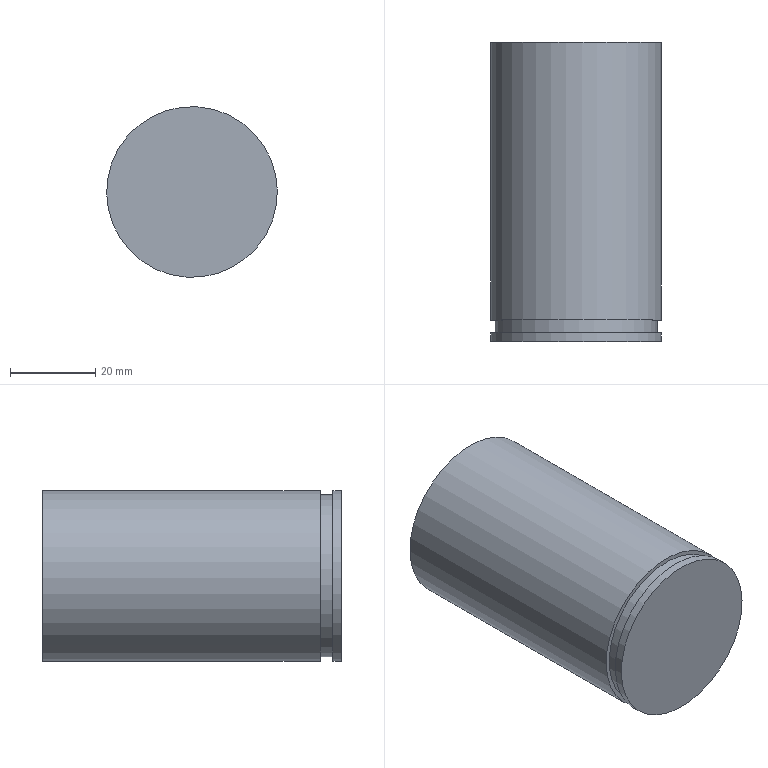Component | NX | MODEL5 | 1 solid | 10 faces | box 40 x 70 x 40 mm | volume 59821 mm3 | cylinder 4 | plane 4 | cone 2 | commonest cylinder face diameters 40 x2 25 x1 38 x1
STEP:
#1=CARTESIAN_POINT('',(0.,0.,0.));
#2=DIRECTION('',(0.,0.,1.));
#3=DIRECTION('',(1.,0.,0.));
#4=AXIS2_PLACEMENT_3D('',#1,#2,#3);
#5=CARTESIAN_POINT('',(18.481,-498.,7.646));
#6=VERTEX_POINT('',#5);
#7=CARTESIAN_POINT('',(-18.481,-498.,-7.646));
#8=VERTEX_POINT('',#7);
#9=CARTESIAN_POINT('',(0.,-498.,0.));
#10=DIRECTION('',(0.,1.,0.));
#11=DIRECTION('',(-0.924,0.,-0.3823));
#12=AXIS2_PLACEMENT_3D('',#9,#10,#11);
#13=CIRCLE('',#12,20.);
#14=CARTESIAN_POINT('',(0.,-568.,0.));
#15=DIRECTION('',(0.,1.,0.));
#16=DIRECTION('',(0.924,0.,0.3823));
#17=AXIS2_PLACEMENT_3D('',#14,#15,#16);
#18=CYLINDRICAL_SURFACE('',#17,20.);
#19=CARTESIAN_POINT('',(-3.142,70.));
#20=DIRECTION('',(1.,0.));
#21=VECTOR('',#20,1.);
#22=LINE('',#19,#21);
#23=(GEOMETRIC_REPRESENTATION_CONTEXT(2)PARAMETRIC_REPRESENTATION_CONTEXT()REPRESENTATION_CONTEXT('',''));
#24=DEFINITIONAL_REPRESENTATION('',(#22),#23);
#25=PCURVE('',#18,#24);
#26=CARTESIAN_POINT('',(0.,-498.,0.));
#27=DIRECTION('',(0.,1.,0.));
#28=DIRECTION('',(0.924,0.,0.3823));
#29=AXIS2_PLACEMENT_3D('',#26,#27,#28);
#30=PLANE('',#29);
#31=CARTESIAN_POINT('',(0.,0.));
#32=DIRECTION('',(-1.,0.));
#33=AXIS2_PLACEMENT_2D('',#31,#32);
#34=CIRCLE('',#33,20.);
#35=(GEOMETRIC_REPRESENTATION_CONTEXT(2)PARAMETRIC_REPRESENTATION_CONTEXT()REPRESENTATION_CONTEXT('',''));
#36=DEFINITIONAL_REPRESENTATION('',(#34),#35);
#37=PCURVE('',#30,#36);
#38=SURFACE_CURVE('',#13,(#25,#37),.PCURVE_S1.);
#39=EDGE_CURVE('',#6,#8,#38,.T.);
#40=ORIENTED_EDGE('',*,*,#39,.F.);
#41=CARTESIAN_POINT('',(18.481,-563.,7.646));
#42=VERTEX_POINT('',#41);
#43=CARTESIAN_POINT('',(18.481,-563.,7.646));
#44=CARTESIAN_POINT('',(18.481,-498.,7.646));
#45=B_SPLINE_CURVE_WITH_KNOTS('',1,(#43,#44),.UNSPECIFIED.,.F.,.F.,(2,2),(5.,70.),.PIECEWISE_BEZIER_KNOTS.);
#46=CARTESIAN_POINT('',(0.,0.));
#47=DIRECTION('',(0.,1.));
#48=VECTOR('',#47,1.);
#49=LINE('',#46,#48);
#50=(GEOMETRIC_REPRESENTATION_CONTEXT(2)PARAMETRIC_REPRESENTATION_CONTEXT()REPRESENTATION_CONTEXT('',''));
#51=DEFINITIONAL_REPRESENTATION('',(#49),#50);
#52=PCURVE('',#18,#51);
#53=CARTESIAN_POINT('',(6.283,0.));
#54=DIRECTION('',(0.,1.));
#55=VECTOR('',#54,1.);
#56=LINE('',#53,#55);
#57=(GEOMETRIC_REPRESENTATION_CONTEXT(2)PARAMETRIC_REPRESENTATION_CONTEXT()REPRESENTATION_CONTEXT('',''));
#58=DEFINITIONAL_REPRESENTATION('',(#56),#57);
#59=PCURVE('',#18,#58);
#60=SEAM_CURVE('',#45,(#52,#59),.PCURVE_S1.);
#61=EDGE_CURVE('',#42,#6,#60,.T.);
#62=ORIENTED_EDGE('',*,*,#61,.F.);
#63=CARTESIAN_POINT('',(0.,-563.,0.));
#64=DIRECTION('',(0.,1.,0.));
#65=DIRECTION('',(0.924,0.,0.3823));
#66=AXIS2_PLACEMENT_3D('',#63,#64,#65);
#67=CIRCLE('',#66,20.);
#68=CARTESIAN_POINT('',(0.,5.));
#69=DIRECTION('',(1.,0.));
#70=VECTOR('',#69,1.);
#71=LINE('',#68,#70);
#72=(GEOMETRIC_REPRESENTATION_CONTEXT(2)PARAMETRIC_REPRESENTATION_CONTEXT()REPRESENTATION_CONTEXT('',''));
#73=DEFINITIONAL_REPRESENTATION('',(#71),#72);
#74=PCURVE('',#18,#73);
#75=CARTESIAN_POINT('',(-18.481,-563.,-7.646));
#76=DIRECTION('',(0.,-1.,0.));
#77=DIRECTION('',(-0.924,0.,-0.3823));
#78=AXIS2_PLACEMENT_3D('',#75,#76,#77);
#79=PLANE('',#78);
#80=CARTESIAN_POINT('',(-40.,-0.));
#81=CARTESIAN_POINT('',(-40.,34.641));
#82=CARTESIAN_POINT('',(-10.,17.321));
#83=CARTESIAN_POINT('',(20.,-0.));
#84=CARTESIAN_POINT('',(-10.,-17.321));
#85=CARTESIAN_POINT('',(-40.,-34.641));
#86=CARTESIAN_POINT('',(-40.,-0.));
#87=(BOUNDED_CURVE()B_SPLINE_CURVE(2,(#80,#81,#82,#83,#84,#85,#86),.UNSPECIFIED.,.T.,.F.)B_SPLINE_CURVE_WITH_KNOTS((1,2,2,2,2,1),(-2.094,0.,2.094,4.189,6.283,8.378),.UNSPECIFIED.)CURVE()GEOMETRIC_REPRESENTATION_ITEM()RATIONAL_B_SPLINE_CURVE((1.,0.5,1.,0.5,1.,0.5,1.))REPRESENTATION_ITEM(''));
#88=(GEOMETRIC_REPRESENTATION_CONTEXT(2)PARAMETRIC_REPRESENTATION_CONTEXT()REPRESENTATION_CONTEXT('',''));
#89=DEFINITIONAL_REPRESENTATION('',(#87),#88);
#90=PCURVE('',#79,#89);
#91=SURFACE_CURVE('',#67,(#74,#90),.PCURVE_S1.);
#92=EDGE_CURVE('',#42,#42,#91,.T.);
#93=ORIENTED_EDGE('',*,*,#92,.T.);
#94=ORIENTED_EDGE('',*,*,#61,.T.);
#95=CARTESIAN_POINT('',(0.,-498.,0.));
#96=DIRECTION('',(0.,1.,0.));
#97=DIRECTION('',(-0.924,0.,-0.3823));
#98=AXIS2_PLACEMENT_3D('',#95,#96,#97);
#99=CIRCLE('',#98,20.);
#100=CARTESIAN_POINT('',(3.142,70.));
#101=DIRECTION('',(1.,0.));
#102=VECTOR('',#101,1.);
#103=LINE('',#100,#102);
#104=(GEOMETRIC_REPRESENTATION_CONTEXT(2)PARAMETRIC_REPRESENTATION_CONTEXT()REPRESENTATION_CONTEXT('',''));
#105=DEFINITIONAL_REPRESENTATION('',(#103),#104);
#106=PCURVE('',#18,#105);
#107=CARTESIAN_POINT('',(0.,0.));
#108=DIRECTION('',(-1.,0.));
#109=AXIS2_PLACEMENT_2D('',#107,#108);
#110=CIRCLE('',#109,20.);
#111=(GEOMETRIC_REPRESENTATION_CONTEXT(2)PARAMETRIC_REPRESENTATION_CONTEXT()REPRESENTATION_CONTEXT('',''));
#112=DEFINITIONAL_REPRESENTATION('',(#110),#111);
#113=PCURVE('',#30,#112);
#114=SURFACE_CURVE('',#99,(#106,#113),.PCURVE_S1.);
#115=EDGE_CURVE('',#8,#6,#114,.T.);
#116=ORIENTED_EDGE('',*,*,#115,.F.);
#117=EDGE_LOOP('',(#40,#62,#93,#94,#116));
#118=FACE_BOUND('',#117,.T.);
#119=ADVANCED_FACE('',(#118),#18,.T.);
#120=CARTESIAN_POINT('',(12.474,-498.,5.161));
#121=VERTEX_POINT('',#120);
#122=CARTESIAN_POINT('',(0.,-498.,0.));
#123=DIRECTION('',(0.,-1.,0.));
#124=DIRECTION('',(0.924,0.,0.3823));
#125=AXIS2_PLACEMENT_3D('',#122,#123,#124);
#126=CIRCLE('',#125,13.5);
#127=CARTESIAN_POINT('',(13.5,0.));
#128=CARTESIAN_POINT('',(13.5,-23.383));
#129=CARTESIAN_POINT('',(-6.75,-11.691));
#130=CARTESIAN_POINT('',(-27.,-0.));
#131=CARTESIAN_POINT('',(-6.75,11.691));
#132=CARTESIAN_POINT('',(13.5,23.383));
#133=CARTESIAN_POINT('',(13.5,0.));
#134=(BOUNDED_CURVE()B_SPLINE_CURVE(2,(#127,#128,#129,#130,#131,#132,#133),.UNSPECIFIED.,.T.,.F.)B_SPLINE_CURVE_WITH_KNOTS((1,2,2,2,2,1),(-2.094,0.,2.094,4.189,6.283,8.378),.UNSPECIFIED.)CURVE()GEOMETRIC_REPRESENTATION_ITEM()RATIONAL_B_SPLINE_CURVE((1.,0.5,1.,0.5,1.,0.5,1.))REPRESENTATION_ITEM(''));
#135=(GEOMETRIC_REPRESENTATION_CONTEXT(2)PARAMETRIC_REPRESENTATION_CONTEXT()REPRESENTATION_CONTEXT('',''));
#136=DEFINITIONAL_REPRESENTATION('',(#134),#135);
#137=PCURVE('',#30,#136);
#138=CARTESIAN_POINT('',(0.,-498.,0.));
#139=DIRECTION('',(0.,1.,0.));
#140=DIRECTION('',(0.924,0.,0.3823));
#141=AXIS2_PLACEMENT_3D('',#138,#139,#140);
#142=CONICAL_SURFACE('',#141,13.5,0.7854);
#143=CARTESIAN_POINT('',(6.283,0.));
#144=DIRECTION('',(-1.,0.));
#145=VECTOR('',#144,1.);
#146=LINE('',#143,#145);
#147=(GEOMETRIC_REPRESENTATION_CONTEXT(2)PARAMETRIC_REPRESENTATION_CONTEXT()REPRESENTATION_CONTEXT('',''));
#148=DEFINITIONAL_REPRESENTATION('',(#146),#147);
#149=PCURVE('',#142,#148);
#150=SURFACE_CURVE('',#126,(#137,#149),.PCURVE_S1.);
#151=EDGE_CURVE('',#121,#121,#150,.T.);
#152=ORIENTED_EDGE('',*,*,#151,.T.);
#153=EDGE_LOOP('',(#152));
#154=FACE_BOUND('',#153,.T.);
#155=ORIENTED_EDGE('',*,*,#115,.T.);
#156=ORIENTED_EDGE('',*,*,#39,.T.);
#157=EDGE_LOOP('',(#155,#156));
#158=FACE_BOUND('',#157,.T.);
#159=ADVANCED_FACE('',(#154,#158),#30,.T.);
#160=CARTESIAN_POINT('',(-11.55,-552.,-4.779));
#161=VERTEX_POINT('',#160);
#162=CARTESIAN_POINT('',(11.55,-552.,4.779));
#163=VERTEX_POINT('',#162);
#164=CARTESIAN_POINT('',(0.,-552.,0.));
#165=DIRECTION('',(0.,-1.,0.));
#166=DIRECTION('',(-0.924,0.,-0.3823));
#167=AXIS2_PLACEMENT_3D('',#164,#165,#166);
#168=CIRCLE('',#167,12.5);
#169=CARTESIAN_POINT('',(0.,-552.,0.));
#170=DIRECTION('',(0.,1.,0.));
#171=DIRECTION('',(0.924,0.,0.3823));
#172=AXIS2_PLACEMENT_3D('',#169,#170,#171);
#173=CONICAL_SURFACE('',#172,12.5,1.03);
#174=CARTESIAN_POINT('',(3.142,0.));
#175=DIRECTION('',(-1.,0.));
#176=VECTOR('',#175,1.);
#177=LINE('',#174,#176);
#178=(GEOMETRIC_REPRESENTATION_CONTEXT(2)PARAMETRIC_REPRESENTATION_CONTEXT()REPRESENTATION_CONTEXT('',''));
#179=DEFINITIONAL_REPRESENTATION('',(#177),#178);
#180=PCURVE('',#173,#179);
#181=CARTESIAN_POINT('',(0.,-498.,0.));
#182=DIRECTION('',(0.,-1.,0.));
#183=DIRECTION('',(-0.924,0.,-0.3823));
#184=AXIS2_PLACEMENT_3D('',#181,#182,#183);
#185=CYLINDRICAL_SURFACE('',#184,12.5);
#186=CARTESIAN_POINT('',(6.283,54.));
#187=DIRECTION('',(1.,0.));
#188=VECTOR('',#187,1.);
#189=LINE('',#186,#188);
#190=(GEOMETRIC_REPRESENTATION_CONTEXT(2)PARAMETRIC_REPRESENTATION_CONTEXT()REPRESENTATION_CONTEXT('',''));
#191=DEFINITIONAL_REPRESENTATION('',(#189),#190);
#192=PCURVE('',#185,#191);
#193=SURFACE_CURVE('',#168,(#180,#192),.PCURVE_S1.);
#194=EDGE_CURVE('',#161,#163,#193,.T.);
#195=ORIENTED_EDGE('',*,*,#194,.T.);
#196=CARTESIAN_POINT('',(0.,-559.511,0.));
#197=VERTEX_POINT('',#196);
#198=CARTESIAN_POINT('',(0.,-559.511,0.));
#199=CARTESIAN_POINT('',(11.55,-552.,4.779));
#200=B_SPLINE_CURVE_WITH_KNOTS('',1,(#198,#199),.UNSPECIFIED.,.F.,.F.,(2,2),(-14.583,0.),.PIECEWISE_BEZIER_KNOTS.);
#201=CARTESIAN_POINT('',(0.,0.));
#202=DIRECTION('',(0.,1.));
#203=VECTOR('',#202,1.);
#204=LINE('',#201,#203);
#205=(GEOMETRIC_REPRESENTATION_CONTEXT(2)PARAMETRIC_REPRESENTATION_CONTEXT()REPRESENTATION_CONTEXT('',''));
#206=DEFINITIONAL_REPRESENTATION('',(#204),#205);
#207=PCURVE('',#173,#206);
#208=CARTESIAN_POINT('',(6.283,0.));
#209=DIRECTION('',(0.,1.));
#210=VECTOR('',#209,1.);
#211=LINE('',#208,#210);
#212=(GEOMETRIC_REPRESENTATION_CONTEXT(2)PARAMETRIC_REPRESENTATION_CONTEXT()REPRESENTATION_CONTEXT('',''));
#213=DEFINITIONAL_REPRESENTATION('',(#211),#212);
#214=PCURVE('',#173,#213);
#215=SEAM_CURVE('',#200,(#207,#214),.PCURVE_S1.);
#216=EDGE_CURVE('',#197,#163,#215,.T.);
#217=ORIENTED_EDGE('',*,*,#216,.F.);
#218=ORIENTED_EDGE('',*,*,#216,.T.);
#219=CARTESIAN_POINT('',(0.,-552.,0.));
#220=DIRECTION('',(0.,-1.,0.));
#221=DIRECTION('',(-0.924,0.,-0.3823));
#222=AXIS2_PLACEMENT_3D('',#219,#220,#221);
#223=CIRCLE('',#222,12.5);
#224=CARTESIAN_POINT('',(9.425,0.));
#225=DIRECTION('',(-1.,0.));
#226=VECTOR('',#225,1.);
#227=LINE('',#224,#226);
#228=(GEOMETRIC_REPRESENTATION_CONTEXT(2)PARAMETRIC_REPRESENTATION_CONTEXT()REPRESENTATION_CONTEXT('',''));
#229=DEFINITIONAL_REPRESENTATION('',(#227),#228);
#230=PCURVE('',#173,#229);
#231=CARTESIAN_POINT('',(0.,54.));
#232=DIRECTION('',(1.,0.));
#233=VECTOR('',#232,1.);
#234=LINE('',#231,#233);
#235=(GEOMETRIC_REPRESENTATION_CONTEXT(2)PARAMETRIC_REPRESENTATION_CONTEXT()REPRESENTATION_CONTEXT('',''));
#236=DEFINITIONAL_REPRESENTATION('',(#234),#235);
#237=PCURVE('',#185,#236);
#238=SURFACE_CURVE('',#223,(#230,#237),.PCURVE_S1.);
#239=EDGE_CURVE('',#163,#161,#238,.T.);
#240=ORIENTED_EDGE('',*,*,#239,.T.);
#241=EDGE_LOOP('',(#195,#217,#218,#240));
#242=FACE_BOUND('',#241,.F.);
#243=ADVANCED_FACE('',(#242),#173,.F.);
#244=CARTESIAN_POINT('',(11.55,-499.,4.779));
#245=VERTEX_POINT('',#244);
#246=CARTESIAN_POINT('',(0.,-499.,0.));
#247=DIRECTION('',(0.,1.,0.));
#248=DIRECTION('',(0.924,0.,0.3823));
#249=AXIS2_PLACEMENT_3D('',#246,#247,#248);
#250=CIRCLE('',#249,12.5);
#251=CARTESIAN_POINT('',(9.425,1.));
#252=DIRECTION('',(-1.,0.));
#253=VECTOR('',#252,1.);
#254=LINE('',#251,#253);
#255=(GEOMETRIC_REPRESENTATION_CONTEXT(2)PARAMETRIC_REPRESENTATION_CONTEXT()REPRESENTATION_CONTEXT('',''));
#256=DEFINITIONAL_REPRESENTATION('',(#254),#255);
#257=PCURVE('',#185,#256);
#258=CARTESIAN_POINT('',(0.,-1.));
#259=DIRECTION('',(1.,-0.));
#260=VECTOR('',#259,1.);
#261=LINE('',#258,#260);
#262=(GEOMETRIC_REPRESENTATION_CONTEXT(2)PARAMETRIC_REPRESENTATION_CONTEXT()REPRESENTATION_CONTEXT('',''));
#263=DEFINITIONAL_REPRESENTATION('',(#261),#262);
#264=PCURVE('',#142,#263);
#265=SURFACE_CURVE('',#250,(#257,#264),.PCURVE_S1.);
#266=EDGE_CURVE('',#245,#245,#265,.T.);
#267=ORIENTED_EDGE('',*,*,#266,.F.);
#268=CARTESIAN_POINT('',(11.55,-499.,4.779));
#269=CARTESIAN_POINT('',(11.55,-552.,4.779));
#270=B_SPLINE_CURVE_WITH_KNOTS('',1,(#268,#269),.UNSPECIFIED.,.F.,.F.,(2,2),(1.,54.),.PIECEWISE_BEZIER_KNOTS.);
#271=CARTESIAN_POINT('',(9.425,0.));
#272=DIRECTION('',(0.,1.));
#273=VECTOR('',#272,1.);
#274=LINE('',#271,#273);
#275=(GEOMETRIC_REPRESENTATION_CONTEXT(2)PARAMETRIC_REPRESENTATION_CONTEXT()REPRESENTATION_CONTEXT('',''));
#276=DEFINITIONAL_REPRESENTATION('',(#274),#275);
#277=PCURVE('',#185,#276);
#278=CARTESIAN_POINT('',(3.142,0.));
#279=DIRECTION('',(0.,1.));
#280=VECTOR('',#279,1.);
#281=LINE('',#278,#280);
#282=(GEOMETRIC_REPRESENTATION_CONTEXT(2)PARAMETRIC_REPRESENTATION_CONTEXT()REPRESENTATION_CONTEXT('',''));
#283=DEFINITIONAL_REPRESENTATION('',(#281),#282);
#284=PCURVE('',#185,#283);
#285=SEAM_CURVE('',#270,(#277,#284),.PCURVE_S1.);
#286=EDGE_CURVE('',#245,#163,#285,.T.);
#287=ORIENTED_EDGE('',*,*,#286,.T.);
#288=ORIENTED_EDGE('',*,*,#194,.F.);
#289=ORIENTED_EDGE('',*,*,#239,.F.);
#290=ORIENTED_EDGE('',*,*,#286,.F.);
#291=EDGE_LOOP('',(#267,#287,#288,#289,#290));
#292=FACE_BOUND('',#291,.F.);
#293=ADVANCED_FACE('',(#292),#185,.F.);
#294=ORIENTED_EDGE('',*,*,#266,.T.);
#295=CARTESIAN_POINT('',(11.55,-499.,4.779));
#296=CARTESIAN_POINT('',(12.474,-498.,5.161));
#297=B_SPLINE_CURVE_WITH_KNOTS('',1,(#295,#296),.UNSPECIFIED.,.F.,.F.,(2,2),(-1.414,0.),.PIECEWISE_BEZIER_KNOTS.);
#298=CARTESIAN_POINT('',(6.283,0.));
#299=DIRECTION('',(0.,1.));
#300=VECTOR('',#299,1.);
#301=LINE('',#298,#300);
#302=(GEOMETRIC_REPRESENTATION_CONTEXT(2)PARAMETRIC_REPRESENTATION_CONTEXT()REPRESENTATION_CONTEXT('',''));
#303=DEFINITIONAL_REPRESENTATION('',(#301),#302);
#304=PCURVE('',#142,#303);
#305=CARTESIAN_POINT('',(0.,0.));
#306=DIRECTION('',(0.,1.));
#307=VECTOR('',#306,1.);
#308=LINE('',#305,#307);
#309=(GEOMETRIC_REPRESENTATION_CONTEXT(2)PARAMETRIC_REPRESENTATION_CONTEXT()REPRESENTATION_CONTEXT('',''));
#310=DEFINITIONAL_REPRESENTATION('',(#308),#309);
#311=PCURVE('',#142,#310);
#312=SEAM_CURVE('',#297,(#304,#311),.PCURVE_S1.);
#313=EDGE_CURVE('',#245,#121,#312,.T.);
#314=ORIENTED_EDGE('',*,*,#313,.T.);
#315=ORIENTED_EDGE('',*,*,#151,.T.);
#316=ORIENTED_EDGE('',*,*,#313,.F.);
#317=EDGE_LOOP('',(#294,#314,#315,#316));
#318=FACE_BOUND('',#317,.F.);
#319=ADVANCED_FACE('',(#318),#142,.F.);
#320=CARTESIAN_POINT('',(17.557,-563.,7.264));
#321=VERTEX_POINT('',#320);
#322=CARTESIAN_POINT('',(0.,-563.,0.));
#323=DIRECTION('',(0.,1.,0.));
#324=DIRECTION('',(0.924,0.,0.3823));
#325=AXIS2_PLACEMENT_3D('',#322,#323,#324);
#326=CIRCLE('',#325,19.);
#327=CARTESIAN_POINT('',(-39.,-0.));
#328=CARTESIAN_POINT('',(-39.,32.909));
#329=CARTESIAN_POINT('',(-10.5,16.454));
#330=CARTESIAN_POINT('',(18.,-0.));
#331=CARTESIAN_POINT('',(-10.5,-16.454));
#332=CARTESIAN_POINT('',(-39.,-32.909));
#333=CARTESIAN_POINT('',(-39.,-0.));
#334=(BOUNDED_CURVE()B_SPLINE_CURVE(2,(#327,#328,#329,#330,#331,#332,#333),.UNSPECIFIED.,.T.,.F.)B_SPLINE_CURVE_WITH_KNOTS((1,2,2,2,2,1),(-2.094,0.,2.094,4.189,6.283,8.378),.UNSPECIFIED.)CURVE()GEOMETRIC_REPRESENTATION_ITEM()RATIONAL_B_SPLINE_CURVE((1.,0.5,1.,0.5,1.,0.5,1.))REPRESENTATION_ITEM(''));
#335=(GEOMETRIC_REPRESENTATION_CONTEXT(2)PARAMETRIC_REPRESENTATION_CONTEXT()REPRESENTATION_CONTEXT('',''));
#336=DEFINITIONAL_REPRESENTATION('',(#334),#335);
#337=PCURVE('',#79,#336);
#338=CARTESIAN_POINT('',(0.,-498.,0.));
#339=DIRECTION('',(0.,1.,0.));
#340=DIRECTION('',(0.924,0.,0.3823));
#341=AXIS2_PLACEMENT_3D('',#338,#339,#340);
#342=CYLINDRICAL_SURFACE('',#341,19.);
#343=CARTESIAN_POINT('',(0.,-65.));
#344=DIRECTION('',(1.,0.));
#345=VECTOR('',#344,1.);
#346=LINE('',#343,#345);
#347=(GEOMETRIC_REPRESENTATION_CONTEXT(2)PARAMETRIC_REPRESENTATION_CONTEXT()REPRESENTATION_CONTEXT('',''));
#348=DEFINITIONAL_REPRESENTATION('',(#346),#347);
#349=PCURVE('',#342,#348);
#350=SURFACE_CURVE('',#326,(#337,#349),.PCURVE_S1.);
#351=EDGE_CURVE('',#321,#321,#350,.T.);
#352=ORIENTED_EDGE('',*,*,#351,.T.);
#353=EDGE_LOOP('',(#352));
#354=FACE_BOUND('',#353,.T.);
#355=ORIENTED_EDGE('',*,*,#92,.F.);
#356=EDGE_LOOP('',(#355));
#357=FACE_BOUND('',#356,.T.);
#358=ADVANCED_FACE('',(#354,#357),#79,.T.);
#359=CARTESIAN_POINT('',(17.557,-566.,7.264));
#360=VERTEX_POINT('',#359);
#361=CARTESIAN_POINT('',(0.,-566.,0.));
#362=DIRECTION('',(0.,1.,0.));
#363=DIRECTION('',(0.924,0.,0.3823));
#364=AXIS2_PLACEMENT_3D('',#361,#362,#363);
#365=CIRCLE('',#364,19.);
#366=CARTESIAN_POINT('',(0.,-68.));
#367=DIRECTION('',(1.,0.));
#368=VECTOR('',#367,1.);
#369=LINE('',#366,#368);
#370=(GEOMETRIC_REPRESENTATION_CONTEXT(2)PARAMETRIC_REPRESENTATION_CONTEXT()REPRESENTATION_CONTEXT('',''));
#371=DEFINITIONAL_REPRESENTATION('',(#369),#370);
#372=PCURVE('',#342,#371);
#373=CARTESIAN_POINT('',(-17.557,-566.,-7.264));
#374=DIRECTION('',(0.,1.,0.));
#375=DIRECTION('',(0.924,0.,0.3823));
#376=AXIS2_PLACEMENT_3D('',#373,#374,#375);
#377=PLANE('',#376);
#378=CARTESIAN_POINT('',(19.,0.));
#379=DIRECTION('',(1.,0.));
#380=AXIS2_PLACEMENT_2D('',#378,#379);
#381=CIRCLE('',#380,19.);
#382=(GEOMETRIC_REPRESENTATION_CONTEXT(2)PARAMETRIC_REPRESENTATION_CONTEXT()REPRESENTATION_CONTEXT('',''));
#383=DEFINITIONAL_REPRESENTATION('',(#381),#382);
#384=PCURVE('',#377,#383);
#385=SURFACE_CURVE('',#365,(#372,#384),.PCURVE_S1.);
#386=EDGE_CURVE('',#360,#360,#385,.T.);
#387=ORIENTED_EDGE('',*,*,#386,.T.);
#388=CARTESIAN_POINT('',(17.557,-566.,7.264));
#389=CARTESIAN_POINT('',(17.557,-563.,7.264));
#390=B_SPLINE_CURVE_WITH_KNOTS('',1,(#388,#389),.UNSPECIFIED.,.F.,.F.,(2,2),(-68.,-65.),.PIECEWISE_BEZIER_KNOTS.);
#391=CARTESIAN_POINT('',(6.283,0.));
#392=DIRECTION('',(0.,1.));
#393=VECTOR('',#392,1.);
#394=LINE('',#391,#393);
#395=(GEOMETRIC_REPRESENTATION_CONTEXT(2)PARAMETRIC_REPRESENTATION_CONTEXT()REPRESENTATION_CONTEXT('',''));
#396=DEFINITIONAL_REPRESENTATION('',(#394),#395);
#397=PCURVE('',#342,#396);
#398=CARTESIAN_POINT('',(0.,0.));
#399=DIRECTION('',(0.,1.));
#400=VECTOR('',#399,1.);
#401=LINE('',#398,#400);
#402=(GEOMETRIC_REPRESENTATION_CONTEXT(2)PARAMETRIC_REPRESENTATION_CONTEXT()REPRESENTATION_CONTEXT('',''));
#403=DEFINITIONAL_REPRESENTATION('',(#401),#402);
#404=PCURVE('',#342,#403);
#405=SEAM_CURVE('',#390,(#397,#404),.PCURVE_S1.);
#406=EDGE_CURVE('',#360,#321,#405,.T.);
#407=ORIENTED_EDGE('',*,*,#406,.T.);
#408=ORIENTED_EDGE('',*,*,#351,.F.);
#409=ORIENTED_EDGE('',*,*,#406,.F.);
#410=EDGE_LOOP('',(#387,#407,#408,#409));
#411=FACE_BOUND('',#410,.T.);
#412=ADVANCED_FACE('',(#411),#342,.T.);
#413=CARTESIAN_POINT('',(18.481,-566.,7.646));
#414=VERTEX_POINT('',#413);
#415=CARTESIAN_POINT('',(0.,-566.,0.));
#416=DIRECTION('',(0.,1.,0.));
#417=DIRECTION('',(0.924,0.,0.3823));
#418=AXIS2_PLACEMENT_3D('',#415,#416,#417);
#419=CIRCLE('',#418,20.);
#420=CARTESIAN_POINT('',(19.,0.));
#421=DIRECTION('',(1.,0.));
#422=AXIS2_PLACEMENT_2D('',#420,#421);
#423=CIRCLE('',#422,20.);
#424=(GEOMETRIC_REPRESENTATION_CONTEXT(2)PARAMETRIC_REPRESENTATION_CONTEXT()REPRESENTATION_CONTEXT('',''));
#425=DEFINITIONAL_REPRESENTATION('',(#423),#424);
#426=PCURVE('',#377,#425);
#427=CARTESIAN_POINT('',(0.,-568.,0.));
#428=DIRECTION('',(0.,1.,0.));
#429=DIRECTION('',(0.924,0.,0.3823));
#430=AXIS2_PLACEMENT_3D('',#427,#428,#429);
#431=CYLINDRICAL_SURFACE('',#430,20.);
#432=CARTESIAN_POINT('',(0.,2.));
#433=DIRECTION('',(1.,0.));
#434=VECTOR('',#433,1.);
#435=LINE('',#432,#434);
#436=(GEOMETRIC_REPRESENTATION_CONTEXT(2)PARAMETRIC_REPRESENTATION_CONTEXT()REPRESENTATION_CONTEXT('',''));
#437=DEFINITIONAL_REPRESENTATION('',(#435),#436);
#438=PCURVE('',#431,#437);
#439=SURFACE_CURVE('',#419,(#426,#438),.PCURVE_S1.);
#440=EDGE_CURVE('',#414,#414,#439,.T.);
#441=ORIENTED_EDGE('',*,*,#440,.T.);
#442=EDGE_LOOP('',(#441));
#443=FACE_BOUND('',#442,.T.);
#444=ORIENTED_EDGE('',*,*,#386,.F.);
#445=EDGE_LOOP('',(#444));
#446=FACE_BOUND('',#445,.T.);
#447=ADVANCED_FACE('',(#443,#446),#377,.T.);
#448=CARTESIAN_POINT('',(-18.481,-568.,-7.646));
#449=VERTEX_POINT('',#448);
#450=CARTESIAN_POINT('',(18.481,-568.,7.646));
#451=VERTEX_POINT('',#450);
#452=CARTESIAN_POINT('',(0.,-568.,0.));
#453=DIRECTION('',(0.,1.,0.));
#454=DIRECTION('',(-0.924,0.,-0.3823));
#455=AXIS2_PLACEMENT_3D('',#452,#453,#454);
#456=CIRCLE('',#455,20.);
#457=CARTESIAN_POINT('',(0.,-568.,0.));
#458=DIRECTION('',(0.,1.,0.));
#459=DIRECTION('',(0.924,0.,0.3823));
#460=AXIS2_PLACEMENT_3D('',#457,#458,#459);
#461=PLANE('',#460);
#462=CARTESIAN_POINT('',(0.,0.));
#463=DIRECTION('',(-1.,0.));
#464=AXIS2_PLACEMENT_2D('',#462,#463);
#465=CIRCLE('',#464,20.);
#466=(GEOMETRIC_REPRESENTATION_CONTEXT(2)PARAMETRIC_REPRESENTATION_CONTEXT()REPRESENTATION_CONTEXT('',''));
#467=DEFINITIONAL_REPRESENTATION('',(#465),#466);
#468=PCURVE('',#461,#467);
#469=CARTESIAN_POINT('',(3.142,0.));
#470=DIRECTION('',(1.,0.));
#471=VECTOR('',#470,1.);
#472=LINE('',#469,#471);
#473=(GEOMETRIC_REPRESENTATION_CONTEXT(2)PARAMETRIC_REPRESENTATION_CONTEXT()REPRESENTATION_CONTEXT('',''));
#474=DEFINITIONAL_REPRESENTATION('',(#472),#473);
#475=PCURVE('',#431,#474);
#476=SURFACE_CURVE('',#456,(#468,#475),.PCURVE_S1.);
#477=EDGE_CURVE('',#449,#451,#476,.T.);
#478=ORIENTED_EDGE('',*,*,#477,.F.);
#479=CARTESIAN_POINT('',(0.,-568.,0.));
#480=DIRECTION('',(0.,1.,0.));
#481=DIRECTION('',(-0.924,0.,-0.3823));
#482=AXIS2_PLACEMENT_3D('',#479,#480,#481);
#483=CIRCLE('',#482,20.);
#484=CARTESIAN_POINT('',(0.,0.));
#485=DIRECTION('',(-1.,0.));
#486=AXIS2_PLACEMENT_2D('',#484,#485);
#487=CIRCLE('',#486,20.);
#488=(GEOMETRIC_REPRESENTATION_CONTEXT(2)PARAMETRIC_REPRESENTATION_CONTEXT()REPRESENTATION_CONTEXT('',''));
#489=DEFINITIONAL_REPRESENTATION('',(#487),#488);
#490=PCURVE('',#461,#489);
#491=CARTESIAN_POINT('',(-3.142,0.));
#492=DIRECTION('',(1.,0.));
#493=VECTOR('',#492,1.);
#494=LINE('',#491,#493);
#495=(GEOMETRIC_REPRESENTATION_CONTEXT(2)PARAMETRIC_REPRESENTATION_CONTEXT()REPRESENTATION_CONTEXT('',''));
#496=DEFINITIONAL_REPRESENTATION('',(#494),#495);
#497=PCURVE('',#431,#496);
#498=SURFACE_CURVE('',#483,(#490,#497),.PCURVE_S1.);
#499=EDGE_CURVE('',#451,#449,#498,.T.);
#500=ORIENTED_EDGE('',*,*,#499,.F.);
#501=EDGE_LOOP('',(#478,#500));
#502=FACE_BOUND('',#501,.T.);
#503=ADVANCED_FACE('',(#502),#461,.F.);
#504=ORIENTED_EDGE('',*,*,#477,.T.);
#505=CARTESIAN_POINT('',(18.481,-568.,7.646));
#506=CARTESIAN_POINT('',(18.481,-566.,7.646));
#507=B_SPLINE_CURVE_WITH_KNOTS('',1,(#505,#506),.UNSPECIFIED.,.F.,.F.,(2,2),(0.,2.),.PIECEWISE_BEZIER_KNOTS.);
#508=CARTESIAN_POINT('',(6.283,0.));
#509=DIRECTION('',(0.,1.));
#510=VECTOR('',#509,1.);
#511=LINE('',#508,#510);
#512=(GEOMETRIC_REPRESENTATION_CONTEXT(2)PARAMETRIC_REPRESENTATION_CONTEXT()REPRESENTATION_CONTEXT('',''));
#513=DEFINITIONAL_REPRESENTATION('',(#511),#512);
#514=PCURVE('',#431,#513);
#515=CARTESIAN_POINT('',(0.,0.));
#516=DIRECTION('',(0.,1.));
#517=VECTOR('',#516,1.);
#518=LINE('',#515,#517);
#519=(GEOMETRIC_REPRESENTATION_CONTEXT(2)PARAMETRIC_REPRESENTATION_CONTEXT()REPRESENTATION_CONTEXT('',''));
#520=DEFINITIONAL_REPRESENTATION('',(#518),#519);
#521=PCURVE('',#431,#520);
#522=SEAM_CURVE('',#507,(#514,#521),.PCURVE_S1.);
#523=EDGE_CURVE('',#451,#414,#522,.T.);
#524=ORIENTED_EDGE('',*,*,#523,.T.);
#525=ORIENTED_EDGE('',*,*,#440,.F.);
#526=ORIENTED_EDGE('',*,*,#523,.F.);
#527=ORIENTED_EDGE('',*,*,#499,.T.);
#528=EDGE_LOOP('',(#504,#524,#525,#526,#527));
#529=FACE_BOUND('',#528,.T.);
#530=ADVANCED_FACE('',(#529),#431,.T.);
#531=CLOSED_SHELL('',(#119,#159,#243,#293,#319,#358,#412,#447,#503,#530));
#532=MANIFOLD_SOLID_BREP('',#531);
#533=(LENGTH_UNIT()NAMED_UNIT(*)SI_UNIT(.MILLI.,.METRE.));
#534=UNCERTAINTY_MEASURE_WITH_UNIT(LENGTH_MEASURE(0.000005),#533,'','');
#535=(NAMED_UNIT(*)PLANE_ANGLE_UNIT()SI_UNIT($,.RADIAN.));
#536=(NAMED_UNIT(*)SI_UNIT($,.STERADIAN.)SOLID_ANGLE_UNIT());
#537=(GEOMETRIC_REPRESENTATION_CONTEXT(3)GLOBAL_UNCERTAINTY_ASSIGNED_CONTEXT((#534))GLOBAL_UNIT_ASSIGNED_CONTEXT((#533,#535,#536))REPRESENTATION_CONTEXT('',''));
#538=ADVANCED_BREP_SHAPE_REPRESENTATION('',(#4,#532),#537);